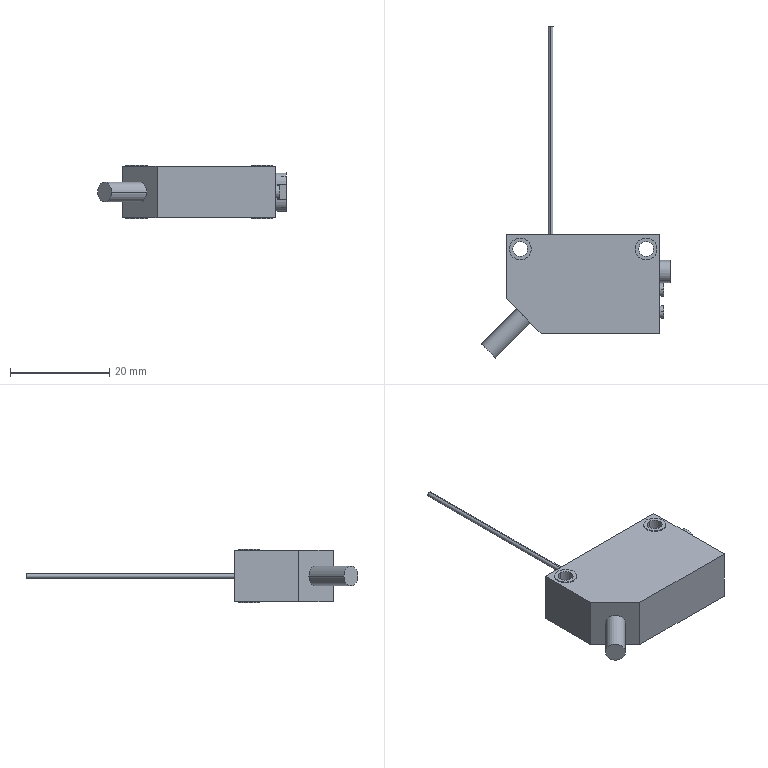Component | SolidWorks | SL010-RightStreamline-1-1_SL010-SensorAssembly-F-1-4_SL010-E3Z_D61-1-1 | 1 solid | 71 faces | volume 6277 mm3 | plane 48 | cylinder 23 | commonest cylinder face diameters 4.4 x8 3 x4 2.6 x4 4.5 x3 1 x2 4 x2